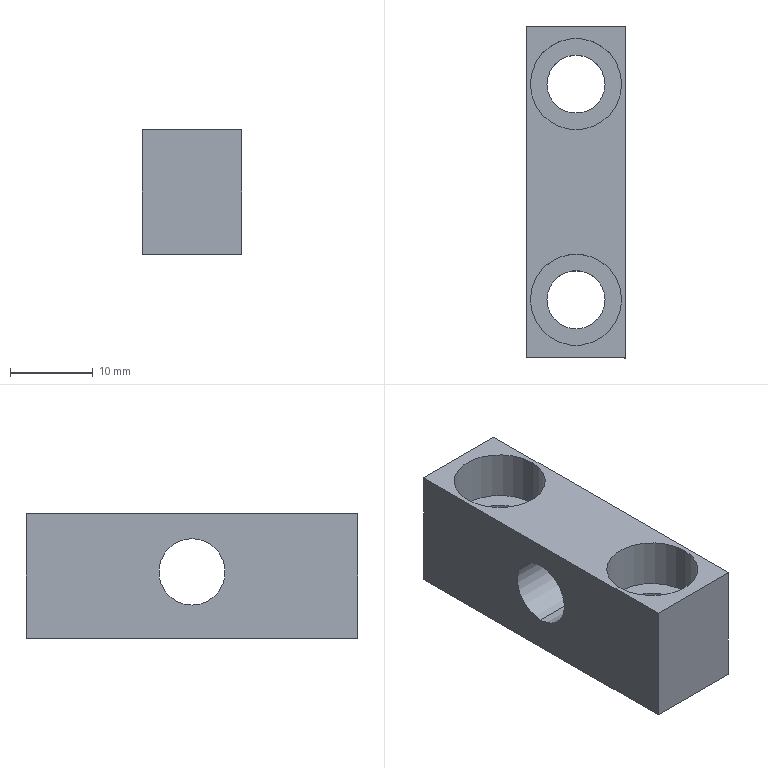Component | SolidWorks | -BeltTensionBlock-1 | 1 solid | 18 faces | box 12 x 40 x 15 mm | volume 4764 mm3 | cylinder 10 | plane 8 | commonest cylinder face diameters 11 x4 7 x4 8 x2
build123d program:
from build123d import *

# Parameters (mm, degrees)
SKETCH1_W                                           = 15
SKETCH1_H                                           = 40
BOSS_EXTRUDE1_DEPTH                                 = 12
SKETCH2_R                                           = 4
CUT_EXTRUDE1_DEPTH                                  = 12
CYLINDRICAL_COUNTERSUNK_HOLE_FOR_M6_HEX_D           = 7
CYLINDRICAL_COUNTERSUNK_HOLE_FOR_M6_HEX_CBORE_D     = 11
CYLINDRICAL_COUNTERSUNK_HOLE_FOR_M6_HEX_CBORE_DEPTH = 6


with BuildPart() as part:
    # Sketch1 → Boss-Extrude1 (new body)
    with BuildSketch(Plane.XY):
        Rectangle(SKETCH1_W, SKETCH1_H)
    extrude(amount=BOSS_EXTRUDE1_DEPTH)

    # Sketch2 → Cut-Extrude1 (cut)
    with BuildSketch(Plane.XY.offset(12)):
        with Locations((0.5, 0)):
            Circle(SKETCH2_R)
    extrude(amount=-CUT_EXTRUDE1_DEPTH, mode=Mode.SUBTRACT)

    # Cylindrical Countersunk Hole for M6 Hex (through all)
    with Locations(Plane(origin=(7.5, 0, 0), x_dir=(0, 0, -1), z_dir=(1, 0, 0))):
        with Locations((-6, 13), (-6, -13)):
            CounterBoreHole(CYLINDRICAL_COUNTERSUNK_HOLE_FOR_M6_HEX_D / 2, CYLINDRICAL_COUNTERSUNK_HOLE_FOR_M6_HEX_CBORE_D / 2, CYLINDRICAL_COUNTERSUNK_HOLE_FOR_M6_HEX_CBORE_DEPTH)


solid = part.part

# Placed as in the assembly
solid = solid.moved(Location((-178, 1094.5, 159.5), (0, -90, 0)))
STEP:
#1=COLOUR_RGB('',0.7922,0.8196,0.9333);
#2=FILL_AREA_STYLE_COLOUR('',#1);
#3=FILL_AREA_STYLE('',(#2));
#4=SURFACE_STYLE_FILL_AREA(#3);
#5=SURFACE_SIDE_STYLE('',(#4));
#6=SURFACE_STYLE_USAGE(.BOTH.,#5);
#7=PRESENTATION_STYLE_ASSIGNMENT((#6));
#8=CARTESIAN_POINT('',(-7.461,43.602,6.339));
#9=VERTEX_POINT('',#8);
#10=CARTESIAN_POINT('',(-7.028,43.602,6.339));
#11=VERTEX_POINT('',#10);
#12=CARTESIAN_POINT('',(-7.244,43.602,6.339));
#13=DIRECTION('',(0.,-0.,1.));
#14=DIRECTION('',(1.,0.,0.));
#15=AXIS2_PLACEMENT_3D('',#12,#13,#14);
#16=CIRCLE('',#15,0.2165);
#17=EDGE_CURVE('',#9,#11,#16,.T.);
#18=ORIENTED_EDGE('',*,*,#17,.F.);
#19=CARTESIAN_POINT('',(-7.461,43.602,6.575));
#20=VERTEX_POINT('',#19);
#21=CARTESIAN_POINT('',(-7.461,43.602,6.575));
#22=DIRECTION('',(0.,-0.,1.));
#23=VECTOR('',#22,39.37);
#24=LINE('',#21,#23);
#25=EDGE_CURVE('',#9,#20,#24,.T.);
#26=ORIENTED_EDGE('',*,*,#25,.T.);
#27=CARTESIAN_POINT('',(-7.028,43.602,6.575));
#28=VERTEX_POINT('',#27);
#29=CARTESIAN_POINT('',(-7.244,43.602,6.575));
#30=DIRECTION('',(0.,-0.,1.));
#31=DIRECTION('',(1.,0.,0.));
#32=AXIS2_PLACEMENT_3D('',#29,#30,#31);
#33=CIRCLE('',#32,0.2165);
#34=EDGE_CURVE('',#20,#28,#33,.T.);
#35=ORIENTED_EDGE('',*,*,#34,.T.);
#36=CARTESIAN_POINT('',(-7.028,43.602,6.575));
#37=DIRECTION('',(0.,-0.,1.));
#38=VECTOR('',#37,39.37);
#39=LINE('',#36,#38);
#40=EDGE_CURVE('',#11,#28,#39,.T.);
#41=ORIENTED_EDGE('',*,*,#40,.F.);
#42=EDGE_LOOP('',(#18,#26,#35,#41));
#43=FACE_OUTER_BOUND('',#42,.T.);
#44=CARTESIAN_POINT('',(-7.244,43.602,6.575));
#45=DIRECTION('',(0.,-0.,1.));
#46=DIRECTION('',(1.,0.,0.));
#47=AXIS2_PLACEMENT_3D('',#44,#45,#46);
#48=CYLINDRICAL_SURFACE('',#47,0.2165);
#49=ADVANCED_FACE('',(#43),#48,.F.);
#50=CARTESIAN_POINT('',(-7.382,43.602,5.984));
#51=VERTEX_POINT('',#50);
#52=CARTESIAN_POINT('',(-7.106,43.602,5.984));
#53=VERTEX_POINT('',#52);
#54=CARTESIAN_POINT('',(-7.244,43.602,5.984));
#55=DIRECTION('',(0.,-0.,1.));
#56=DIRECTION('',(1.,0.,0.));
#57=AXIS2_PLACEMENT_3D('',#54,#55,#56);
#58=CIRCLE('',#57,0.1378);
#59=EDGE_CURVE('',#51,#53,#58,.T.);
#60=ORIENTED_EDGE('',*,*,#59,.F.);
#61=CARTESIAN_POINT('',(-7.382,43.602,6.339));
#62=VERTEX_POINT('',#61);
#63=CARTESIAN_POINT('',(-7.382,43.602,6.575));
#64=DIRECTION('',(0.,-0.,1.));
#65=VECTOR('',#64,39.37);
#66=LINE('',#63,#65);
#67=EDGE_CURVE('',#51,#62,#66,.T.);
#68=ORIENTED_EDGE('',*,*,#67,.T.);
#69=CARTESIAN_POINT('',(-7.106,43.602,6.339));
#70=VERTEX_POINT('',#69);
#71=CARTESIAN_POINT('',(-7.244,43.602,6.339));
#72=DIRECTION('',(0.,-0.,1.));
#73=DIRECTION('',(1.,0.,0.));
#74=AXIS2_PLACEMENT_3D('',#71,#72,#73);
#75=CIRCLE('',#74,0.1378);
#76=EDGE_CURVE('',#62,#70,#75,.T.);
#77=ORIENTED_EDGE('',*,*,#76,.T.);
#78=CARTESIAN_POINT('',(-7.106,43.602,6.575));
#79=DIRECTION('',(0.,-0.,1.));
#80=VECTOR('',#79,39.37);
#81=LINE('',#78,#80);
#82=EDGE_CURVE('',#53,#70,#81,.T.);
#83=ORIENTED_EDGE('',*,*,#82,.F.);
#84=EDGE_LOOP('',(#60,#68,#77,#83));
#85=FACE_OUTER_BOUND('',#84,.T.);
#86=CARTESIAN_POINT('',(-7.244,43.602,6.575));
#87=DIRECTION('',(0.,-0.,1.));
#88=DIRECTION('',(1.,0.,0.));
#89=AXIS2_PLACEMENT_3D('',#86,#87,#88);
#90=CYLINDRICAL_SURFACE('',#89,0.1378);
#91=ADVANCED_FACE('',(#85),#90,.F.);
#92=CARTESIAN_POINT('',(-7.461,42.579,6.339));
#93=VERTEX_POINT('',#92);
#94=CARTESIAN_POINT('',(-7.028,42.579,6.339));
#95=VERTEX_POINT('',#94);
#96=CARTESIAN_POINT('',(-7.244,42.579,6.339));
#97=DIRECTION('',(0.,-0.,1.));
#98=DIRECTION('',(1.,0.,0.));
#99=AXIS2_PLACEMENT_3D('',#96,#97,#98);
#100=CIRCLE('',#99,0.2165);
#101=EDGE_CURVE('',#93,#95,#100,.T.);
#102=ORIENTED_EDGE('',*,*,#101,.F.);
#103=CARTESIAN_POINT('',(-7.461,42.579,6.575));
#104=VERTEX_POINT('',#103);
#105=CARTESIAN_POINT('',(-7.461,42.579,6.575));
#106=DIRECTION('',(0.,-0.,1.));
#107=VECTOR('',#106,39.37);
#108=LINE('',#105,#107);
#109=EDGE_CURVE('',#93,#104,#108,.T.);
#110=ORIENTED_EDGE('',*,*,#109,.T.);
#111=CARTESIAN_POINT('',(-7.028,42.579,6.575));
#112=VERTEX_POINT('',#111);
#113=CARTESIAN_POINT('',(-7.244,42.579,6.575));
#114=DIRECTION('',(0.,-0.,1.));
#115=DIRECTION('',(1.,0.,0.));
#116=AXIS2_PLACEMENT_3D('',#113,#114,#115);
#117=CIRCLE('',#116,0.2165);
#118=EDGE_CURVE('',#104,#112,#117,.T.);
#119=ORIENTED_EDGE('',*,*,#118,.T.);
#120=CARTESIAN_POINT('',(-7.028,42.579,6.575));
#121=DIRECTION('',(0.,-0.,1.));
#122=VECTOR('',#121,39.37);
#123=LINE('',#120,#122);
#124=EDGE_CURVE('',#95,#112,#123,.T.);
#125=ORIENTED_EDGE('',*,*,#124,.F.);
#126=EDGE_LOOP('',(#102,#110,#119,#125));
#127=FACE_OUTER_BOUND('',#126,.T.);
#128=CARTESIAN_POINT('',(-7.244,42.579,6.575));
#129=DIRECTION('',(0.,-0.,1.));
#130=DIRECTION('',(1.,0.,0.));
#131=AXIS2_PLACEMENT_3D('',#128,#129,#130);
#132=CYLINDRICAL_SURFACE('',#131,0.2165);
#133=ADVANCED_FACE('',(#127),#132,.F.);
#134=CARTESIAN_POINT('',(-7.382,42.579,5.984));
#135=VERTEX_POINT('',#134);
#136=CARTESIAN_POINT('',(-7.106,42.579,5.984));
#137=VERTEX_POINT('',#136);
#138=CARTESIAN_POINT('',(-7.244,42.579,5.984));
#139=DIRECTION('',(0.,-0.,1.));
#140=DIRECTION('',(1.,0.,0.));
#141=AXIS2_PLACEMENT_3D('',#138,#139,#140);
#142=CIRCLE('',#141,0.1378);
#143=EDGE_CURVE('',#135,#137,#142,.T.);
#144=ORIENTED_EDGE('',*,*,#143,.F.);
#145=CARTESIAN_POINT('',(-7.382,42.579,6.339));
#146=VERTEX_POINT('',#145);
#147=CARTESIAN_POINT('',(-7.382,42.579,6.575));
#148=DIRECTION('',(0.,-0.,1.));
#149=VECTOR('',#148,39.37);
#150=LINE('',#147,#149);
#151=EDGE_CURVE('',#135,#146,#150,.T.);
#152=ORIENTED_EDGE('',*,*,#151,.T.);
#153=CARTESIAN_POINT('',(-7.106,42.579,6.339));
#154=VERTEX_POINT('',#153);
#155=CARTESIAN_POINT('',(-7.244,42.579,6.339));
#156=DIRECTION('',(0.,-0.,1.));
#157=DIRECTION('',(1.,0.,0.));
#158=AXIS2_PLACEMENT_3D('',#155,#156,#157);
#159=CIRCLE('',#158,0.1378);
#160=EDGE_CURVE('',#146,#154,#159,.T.);
#161=ORIENTED_EDGE('',*,*,#160,.T.);
#162=CARTESIAN_POINT('',(-7.106,42.579,6.575));
#163=DIRECTION('',(0.,-0.,1.));
#164=VECTOR('',#163,39.37);
#165=LINE('',#162,#164);
#166=EDGE_CURVE('',#137,#154,#165,.T.);
#167=ORIENTED_EDGE('',*,*,#166,.F.);
#168=EDGE_LOOP('',(#144,#152,#161,#167));
#169=FACE_OUTER_BOUND('',#168,.T.);
#170=CARTESIAN_POINT('',(-7.244,42.579,6.575));
#171=DIRECTION('',(0.,-0.,1.));
#172=DIRECTION('',(1.,0.,0.));
#173=AXIS2_PLACEMENT_3D('',#170,#171,#172);
#174=CYLINDRICAL_SURFACE('',#173,0.1378);
#175=ADVANCED_FACE('',(#169),#174,.F.);
#176=CARTESIAN_POINT('',(-7.008,43.091,6.142));
#177=VERTEX_POINT('',#176);
#178=CARTESIAN_POINT('',(-7.008,43.091,6.457));
#179=VERTEX_POINT('',#178);
#180=CARTESIAN_POINT('',(-7.008,43.091,6.299));
#181=DIRECTION('',(-1.,0.,0.));
#182=DIRECTION('',(0.,0.,1.));
#183=AXIS2_PLACEMENT_3D('',#180,#181,#182);
#184=CIRCLE('',#183,0.1575);
#185=EDGE_CURVE('',#177,#179,#184,.T.);
#186=ORIENTED_EDGE('',*,*,#185,.F.);
#187=CARTESIAN_POINT('',(-7.48,43.091,6.142));
#188=VERTEX_POINT('',#187);
#189=CARTESIAN_POINT('',(-7.008,43.091,6.142));
#190=DIRECTION('',(-1.,0.,0.));
#191=VECTOR('',#190,39.37);
#192=LINE('',#189,#191);
#193=EDGE_CURVE('',#177,#188,#192,.T.);
#194=ORIENTED_EDGE('',*,*,#193,.T.);
#195=CARTESIAN_POINT('',(-7.48,43.091,6.457));
#196=VERTEX_POINT('',#195);
#197=CARTESIAN_POINT('',(-7.48,43.091,6.299));
#198=DIRECTION('',(-1.,0.,0.));
#199=DIRECTION('',(0.,0.,1.));
#200=AXIS2_PLACEMENT_3D('',#197,#198,#199);
#201=CIRCLE('',#200,0.1575);
#202=EDGE_CURVE('',#188,#196,#201,.T.);
#203=ORIENTED_EDGE('',*,*,#202,.T.);
#204=CARTESIAN_POINT('',(-7.008,43.091,6.457));
#205=DIRECTION('',(-1.,0.,0.));
#206=VECTOR('',#205,39.37);
#207=LINE('',#204,#206);
#208=EDGE_CURVE('',#179,#196,#207,.T.);
#209=ORIENTED_EDGE('',*,*,#208,.F.);
#210=EDGE_LOOP('',(#186,#194,#203,#209));
#211=FACE_OUTER_BOUND('',#210,.T.);
#212=CARTESIAN_POINT('',(-7.008,43.091,6.299));
#213=DIRECTION('',(-1.,0.,0.));
#214=DIRECTION('',(0.,0.,1.));
#215=AXIS2_PLACEMENT_3D('',#212,#213,#214);
#216=CYLINDRICAL_SURFACE('',#215,0.1575);
#217=ADVANCED_FACE('',(#211),#216,.F.);
#218=CARTESIAN_POINT('',(-7.244,43.602,6.575));
#219=DIRECTION('',(0.,-0.,1.));
#220=DIRECTION('',(1.,0.,0.));
#221=AXIS2_PLACEMENT_3D('',#218,#219,#220);
#222=CIRCLE('',#221,0.2165);
#223=EDGE_CURVE('',#28,#20,#222,.T.);
#224=ORIENTED_EDGE('',*,*,#223,.F.);
#225=ORIENTED_EDGE('',*,*,#34,.F.);
#226=EDGE_LOOP('',(#224,#225));
#227=FACE_BOUND('',#226,.T.);
#228=CARTESIAN_POINT('',(-7.244,42.579,6.575));
#229=DIRECTION('',(0.,-0.,1.));
#230=DIRECTION('',(1.,0.,0.));
#231=AXIS2_PLACEMENT_3D('',#228,#229,#230);
#232=CIRCLE('',#231,0.2165);
#233=EDGE_CURVE('',#112,#104,#232,.T.);
#234=ORIENTED_EDGE('',*,*,#233,.F.);
#235=ORIENTED_EDGE('',*,*,#118,.F.);
#236=EDGE_LOOP('',(#234,#235));
#237=FACE_BOUND('',#236,.T.);
#238=CARTESIAN_POINT('',(-7.008,42.303,6.575));
#239=VERTEX_POINT('',#238);
#240=CARTESIAN_POINT('',(-7.008,43.878,6.575));
#241=VERTEX_POINT('',#240);
#242=CARTESIAN_POINT('',(-7.008,43.878,6.575));
#243=DIRECTION('',(0.,1.,0.));
#244=VECTOR('',#243,39.37);
#245=LINE('',#242,#244);
#246=EDGE_CURVE('',#239,#241,#245,.T.);
#247=ORIENTED_EDGE('',*,*,#246,.T.);
#248=CARTESIAN_POINT('',(-7.48,43.878,6.575));
#249=VERTEX_POINT('',#248);
#250=CARTESIAN_POINT('',(-7.48,43.878,6.575));
#251=DIRECTION('',(1.,-0.,-0.));
#252=VECTOR('',#251,39.37);
#253=LINE('',#250,#252);
#254=EDGE_CURVE('',#249,#241,#253,.T.);
#255=ORIENTED_EDGE('',*,*,#254,.F.);
#256=CARTESIAN_POINT('',(-7.48,42.303,6.575));
#257=VERTEX_POINT('',#256);
#258=CARTESIAN_POINT('',(-7.48,43.878,6.575));
#259=DIRECTION('',(0.,1.,0.));
#260=VECTOR('',#259,39.37);
#261=LINE('',#258,#260);
#262=EDGE_CURVE('',#257,#249,#261,.T.);
#263=ORIENTED_EDGE('',*,*,#262,.F.);
#264=CARTESIAN_POINT('',(-7.48,42.303,6.575));
#265=DIRECTION('',(1.,-0.,-0.));
#266=VECTOR('',#265,39.37);
#267=LINE('',#264,#266);
#268=EDGE_CURVE('',#257,#239,#267,.T.);
#269=ORIENTED_EDGE('',*,*,#268,.T.);
#270=EDGE_LOOP('',(#247,#255,#263,#269));
#271=FACE_OUTER_BOUND('',#270,.T.);
#272=CARTESIAN_POINT('',(-7.48,43.878,6.575));
#273=DIRECTION('',(-0.,0.,-1.));
#274=DIRECTION('',(-0.,-1.,-0.));
#275=AXIS2_PLACEMENT_3D('',#272,#273,#274);
#276=PLANE('',#275);
#277=ADVANCED_FACE('',(#227,#237,#271),#276,.F.);
#278=CARTESIAN_POINT('',(-7.008,43.878,5.984));
#279=VERTEX_POINT('',#278);
#280=CARTESIAN_POINT('',(-7.008,43.878,5.984));
#281=DIRECTION('',(-0.,0.,-1.));
#282=VECTOR('',#281,39.37);
#283=LINE('',#280,#282);
#284=EDGE_CURVE('',#241,#279,#283,.T.);
#285=ORIENTED_EDGE('',*,*,#284,.T.);
#286=CARTESIAN_POINT('',(-7.48,43.878,5.984));
#287=VERTEX_POINT('',#286);
#288=CARTESIAN_POINT('',(-7.48,43.878,5.984));
#289=DIRECTION('',(1.,-0.,-0.));
#290=VECTOR('',#289,39.37);
#291=LINE('',#288,#290);
#292=EDGE_CURVE('',#287,#279,#291,.T.);
#293=ORIENTED_EDGE('',*,*,#292,.F.);
#294=CARTESIAN_POINT('',(-7.48,43.878,5.984));
#295=DIRECTION('',(-0.,0.,-1.));
#296=VECTOR('',#295,39.37);
#297=LINE('',#294,#296);
#298=EDGE_CURVE('',#249,#287,#297,.T.);
#299=ORIENTED_EDGE('',*,*,#298,.F.);
#300=ORIENTED_EDGE('',*,*,#254,.T.);
#301=EDGE_LOOP('',(#285,#293,#299,#300));
#302=FACE_OUTER_BOUND('',#301,.T.);
#303=CARTESIAN_POINT('',(-7.48,43.878,5.984));
#304=DIRECTION('',(-0.,-1.,-0.));
#305=DIRECTION('',(1.,-0.,-0.));
#306=AXIS2_PLACEMENT_3D('',#303,#304,#305);
#307=PLANE('',#306);
#308=ADVANCED_FACE('',(#302),#307,.F.);
#309=CARTESIAN_POINT('',(-7.244,43.602,5.984));
#310=DIRECTION('',(0.,-0.,1.));
#311=DIRECTION('',(1.,0.,0.));
#312=AXIS2_PLACEMENT_3D('',#309,#310,#311);
#313=CIRCLE('',#312,0.1378);
#314=EDGE_CURVE('',#53,#51,#313,.T.);
#315=ORIENTED_EDGE('',*,*,#314,.T.);
#316=ORIENTED_EDGE('',*,*,#59,.T.);
#317=EDGE_LOOP('',(#315,#316));
#318=FACE_BOUND('',#317,.T.);
#319=CARTESIAN_POINT('',(-7.244,42.579,5.984));
#320=DIRECTION('',(0.,-0.,1.));
#321=DIRECTION('',(1.,0.,0.));
#322=AXIS2_PLACEMENT_3D('',#319,#320,#321);
#323=CIRCLE('',#322,0.1378);
#324=EDGE_CURVE('',#137,#135,#323,.T.);
#325=ORIENTED_EDGE('',*,*,#324,.T.);
#326=ORIENTED_EDGE('',*,*,#143,.T.);
#327=EDGE_LOOP('',(#325,#326));
#328=FACE_BOUND('',#327,.T.);
#329=CARTESIAN_POINT('',(-7.008,42.303,5.984));
#330=VERTEX_POINT('',#329);
#331=CARTESIAN_POINT('',(-7.008,43.878,5.984));
#332=DIRECTION('',(-0.,-1.,-0.));
#333=VECTOR('',#332,39.37);
#334=LINE('',#331,#333);
#335=EDGE_CURVE('',#279,#330,#334,.T.);
#336=ORIENTED_EDGE('',*,*,#335,.T.);
#337=CARTESIAN_POINT('',(-7.48,42.303,5.984));
#338=VERTEX_POINT('',#337);
#339=CARTESIAN_POINT('',(-7.48,42.303,5.984));
#340=DIRECTION('',(1.,-0.,-0.));
#341=VECTOR('',#340,39.37);
#342=LINE('',#339,#341);
#343=EDGE_CURVE('',#338,#330,#342,.T.);
#344=ORIENTED_EDGE('',*,*,#343,.F.);
#345=CARTESIAN_POINT('',(-7.48,43.878,5.984));
#346=DIRECTION('',(-0.,-1.,-0.));
#347=VECTOR('',#346,39.37);
#348=LINE('',#345,#347);
#349=EDGE_CURVE('',#287,#338,#348,.T.);
#350=ORIENTED_EDGE('',*,*,#349,.F.);
#351=ORIENTED_EDGE('',*,*,#292,.T.);
#352=EDGE_LOOP('',(#336,#344,#350,#351));
#353=FACE_OUTER_BOUND('',#352,.T.);
#354=CARTESIAN_POINT('',(-7.48,43.878,5.984));
#355=DIRECTION('',(0.,-0.,1.));
#356=DIRECTION('',(0.,1.,0.));
#357=AXIS2_PLACEMENT_3D('',#354,#355,#356);
#358=PLANE('',#357);
#359=ADVANCED_FACE('',(#318,#328,#353),#358,.F.);
#360=CARTESIAN_POINT('',(-7.008,42.303,5.984));
#361=DIRECTION('',(0.,-0.,1.));
#362=VECTOR('',#361,39.37);
#363=LINE('',#360,#362);
#364=EDGE_CURVE('',#330,#239,#363,.T.);
#365=ORIENTED_EDGE('',*,*,#364,.T.);
#366=ORIENTED_EDGE('',*,*,#268,.F.);
#367=CARTESIAN_POINT('',(-7.48,42.303,5.984));
#368=DIRECTION('',(0.,-0.,1.));
#369=VECTOR('',#368,39.37);
#370=LINE('',#367,#369);
#371=EDGE_CURVE('',#338,#257,#370,.T.);
#372=ORIENTED_EDGE('',*,*,#371,.F.);
#373=ORIENTED_EDGE('',*,*,#343,.T.);
#374=EDGE_LOOP('',(#365,#366,#372,#373));
#375=FACE_OUTER_BOUND('',#374,.T.);
#376=CARTESIAN_POINT('',(-7.48,42.303,5.984));
#377=DIRECTION('',(0.,1.,0.));
#378=DIRECTION('',(-1.,0.,0.));
#379=AXIS2_PLACEMENT_3D('',#376,#377,#378);
#380=PLANE('',#379);
#381=ADVANCED_FACE('',(#375),#380,.F.);
#382=CARTESIAN_POINT('',(-7.48,43.091,6.299));
#383=DIRECTION('',(-1.,0.,0.));
#384=DIRECTION('',(0.,0.,1.));
#385=AXIS2_PLACEMENT_3D('',#382,#383,#384);
#386=CIRCLE('',#385,0.1575);
#387=EDGE_CURVE('',#196,#188,#386,.T.);
#388=ORIENTED_EDGE('',*,*,#387,.F.);
#389=ORIENTED_EDGE('',*,*,#202,.F.);
#390=EDGE_LOOP('',(#388,#389));
#391=FACE_BOUND('',#390,.T.);
#392=ORIENTED_EDGE('',*,*,#262,.T.);
#393=ORIENTED_EDGE('',*,*,#298,.T.);
#394=ORIENTED_EDGE('',*,*,#349,.T.);
#395=ORIENTED_EDGE('',*,*,#371,.T.);
#396=EDGE_LOOP('',(#392,#393,#394,#395));
#397=FACE_OUTER_BOUND('',#396,.T.);
#398=CARTESIAN_POINT('',(-7.48,43.091,6.28));
#399=DIRECTION('',(-1.,0.,0.));
#400=DIRECTION('',(0.,-0.,1.));
#401=AXIS2_PLACEMENT_3D('',#398,#399,#400);
#402=PLANE('',#401);
#403=ADVANCED_FACE('',(#391,#397),#402,.T.);
#404=CARTESIAN_POINT('',(-7.008,43.091,6.299));
#405=DIRECTION('',(-1.,0.,0.));
#406=DIRECTION('',(0.,0.,1.));
#407=AXIS2_PLACEMENT_3D('',#404,#405,#406);
#408=CIRCLE('',#407,0.1575);
#409=EDGE_CURVE('',#179,#177,#408,.T.);
#410=ORIENTED_EDGE('',*,*,#409,.T.);
#411=ORIENTED_EDGE('',*,*,#185,.T.);
#412=EDGE_LOOP('',(#410,#411));
#413=FACE_BOUND('',#412,.T.);
#414=ORIENTED_EDGE('',*,*,#246,.F.);
#415=ORIENTED_EDGE('',*,*,#364,.F.);
#416=ORIENTED_EDGE('',*,*,#335,.F.);
#417=ORIENTED_EDGE('',*,*,#284,.F.);
#418=EDGE_LOOP('',(#414,#415,#416,#417));
#419=FACE_OUTER_BOUND('',#418,.T.);
#420=CARTESIAN_POINT('',(-7.008,43.091,6.28));
#421=DIRECTION('',(-1.,0.,0.));
#422=DIRECTION('',(0.,-0.,1.));
#423=AXIS2_PLACEMENT_3D('',#420,#421,#422);
#424=PLANE('',#423);
#425=ADVANCED_FACE('',(#413,#419),#424,.F.);
#426=ORIENTED_EDGE('',*,*,#193,.F.);
#427=ORIENTED_EDGE('',*,*,#409,.F.);
#428=ORIENTED_EDGE('',*,*,#208,.T.);
#429=ORIENTED_EDGE('',*,*,#387,.T.);
#430=EDGE_LOOP('',(#426,#427,#428,#429));
#431=FACE_OUTER_BOUND('',#430,.T.);
#432=CARTESIAN_POINT('',(-7.008,43.091,6.299));
#433=DIRECTION('',(-1.,0.,0.));
#434=DIRECTION('',(0.,0.,1.));
#435=AXIS2_PLACEMENT_3D('',#432,#433,#434);
#436=CYLINDRICAL_SURFACE('',#435,0.1575);
#437=ADVANCED_FACE('',(#431),#436,.F.);
#438=ORIENTED_EDGE('',*,*,#151,.F.);
#439=ORIENTED_EDGE('',*,*,#324,.F.);
#440=ORIENTED_EDGE('',*,*,#166,.T.);
#441=CARTESIAN_POINT('',(-7.244,42.579,6.339));
#442=DIRECTION('',(0.,-0.,1.));
#443=DIRECTION('',(1.,0.,0.));
#444=AXIS2_PLACEMENT_3D('',#441,#442,#443);
#445=CIRCLE('',#444,0.1378);
#446=EDGE_CURVE('',#154,#146,#445,.T.);
#447=ORIENTED_EDGE('',*,*,#446,.T.);
#448=EDGE_LOOP('',(#438,#439,#440,#447));
#449=FACE_OUTER_BOUND('',#448,.T.);
#450=CARTESIAN_POINT('',(-7.244,42.579,6.575));
#451=DIRECTION('',(0.,-0.,1.));
#452=DIRECTION('',(1.,0.,0.));
#453=AXIS2_PLACEMENT_3D('',#450,#451,#452);
#454=CYLINDRICAL_SURFACE('',#453,0.1378);
#455=ADVANCED_FACE('',(#449),#454,.F.);
#456=ORIENTED_EDGE('',*,*,#446,.F.);
#457=ORIENTED_EDGE('',*,*,#160,.F.);
#458=EDGE_LOOP('',(#456,#457));
#459=FACE_BOUND('',#458,.T.);
#460=CARTESIAN_POINT('',(-7.244,42.579,6.339));
#461=DIRECTION('',(0.,-0.,1.));
#462=DIRECTION('',(1.,0.,0.));
#463=AXIS2_PLACEMENT_3D('',#460,#461,#462);
#464=CIRCLE('',#463,0.2165);
#465=EDGE_CURVE('',#95,#93,#464,.T.);
#466=ORIENTED_EDGE('',*,*,#465,.T.);
#467=ORIENTED_EDGE('',*,*,#101,.T.);
#468=EDGE_LOOP('',(#466,#467));
#469=FACE_OUTER_BOUND('',#468,.T.);
#470=CARTESIAN_POINT('',(-7.244,42.717,6.339));
#471=DIRECTION('',(0.,0.,-1.));
#472=DIRECTION('',(-1.,0.,0.));
#473=AXIS2_PLACEMENT_3D('',#470,#471,#472);
#474=PLANE('',#473);
#475=ADVANCED_FACE('',(#459,#469),#474,.F.);
#476=ORIENTED_EDGE('',*,*,#109,.F.);
#477=ORIENTED_EDGE('',*,*,#465,.F.);
#478=ORIENTED_EDGE('',*,*,#124,.T.);
#479=ORIENTED_EDGE('',*,*,#233,.T.);
#480=EDGE_LOOP('',(#476,#477,#478,#479));
#481=FACE_OUTER_BOUND('',#480,.T.);
#482=CARTESIAN_POINT('',(-7.244,42.579,6.575));
#483=DIRECTION('',(0.,-0.,1.));
#484=DIRECTION('',(1.,0.,0.));
#485=AXIS2_PLACEMENT_3D('',#482,#483,#484);
#486=CYLINDRICAL_SURFACE('',#485,0.2165);
#487=ADVANCED_FACE('',(#481),#486,.F.);
#488=ORIENTED_EDGE('',*,*,#67,.F.);
#489=ORIENTED_EDGE('',*,*,#314,.F.);
#490=ORIENTED_EDGE('',*,*,#82,.T.);
#491=CARTESIAN_POINT('',(-7.244,43.602,6.339));
#492=DIRECTION('',(0.,-0.,1.));
#493=DIRECTION('',(1.,0.,0.));
#494=AXIS2_PLACEMENT_3D('',#491,#492,#493);
#495=CIRCLE('',#494,0.1378);
#496=EDGE_CURVE('',#70,#62,#495,.T.);
#497=ORIENTED_EDGE('',*,*,#496,.T.);
#498=EDGE_LOOP('',(#488,#489,#490,#497));
#499=FACE_OUTER_BOUND('',#498,.T.);
#500=CARTESIAN_POINT('',(-7.244,43.602,6.575));
#501=DIRECTION('',(0.,-0.,1.));
#502=DIRECTION('',(1.,0.,0.));
#503=AXIS2_PLACEMENT_3D('',#500,#501,#502);
#504=CYLINDRICAL_SURFACE('',#503,0.1378);
#505=ADVANCED_FACE('',(#499),#504,.F.);
#506=ORIENTED_EDGE('',*,*,#496,.F.);
#507=ORIENTED_EDGE('',*,*,#76,.F.);
#508=EDGE_LOOP('',(#506,#507));
#509=FACE_BOUND('',#508,.T.);
#510=CARTESIAN_POINT('',(-7.244,43.602,6.339));
#511=DIRECTION('',(0.,-0.,1.));
#512=DIRECTION('',(1.,0.,0.));
#513=AXIS2_PLACEMENT_3D('',#510,#511,#512);
#514=CIRCLE('',#513,0.2165);
#515=EDGE_CURVE('',#11,#9,#514,.T.);
#516=ORIENTED_EDGE('',*,*,#515,.T.);
#517=ORIENTED_EDGE('',*,*,#17,.T.);
#518=EDGE_LOOP('',(#516,#517));
#519=FACE_OUTER_BOUND('',#518,.T.);
#520=CARTESIAN_POINT('',(-7.244,43.74,6.339));
#521=DIRECTION('',(0.,0.,-1.));
#522=DIRECTION('',(-1.,0.,0.));
#523=AXIS2_PLACEMENT_3D('',#520,#521,#522);
#524=PLANE('',#523);
#525=ADVANCED_FACE('',(#509,#519),#524,.F.);
#526=ORIENTED_EDGE('',*,*,#25,.F.);
#527=ORIENTED_EDGE('',*,*,#515,.F.);
#528=ORIENTED_EDGE('',*,*,#40,.T.);
#529=ORIENTED_EDGE('',*,*,#223,.T.);
#530=EDGE_LOOP('',(#526,#527,#528,#529));
#531=FACE_OUTER_BOUND('',#530,.T.);
#532=CARTESIAN_POINT('',(-7.244,43.602,6.575));
#533=DIRECTION('',(0.,-0.,1.));
#534=DIRECTION('',(1.,0.,0.));
#535=AXIS2_PLACEMENT_3D('',#532,#533,#534);
#536=CYLINDRICAL_SURFACE('',#535,0.2165);
#537=ADVANCED_FACE('',(#531),#536,.F.);
#538=CLOSED_SHELL('',(#49,#91,#133,#175,#217,#277,#308,#359,#381,#403,#425,#437,#455,#475,#487,#505,#525,#537));
#539=MANIFOLD_SOLID_BREP('',#538);
#540=STYLED_ITEM('',(#7),#539);
#541=(LENGTH_UNIT()NAMED_UNIT(*)SI_UNIT($,.METRE.));
#542=LENGTH_MEASURE_WITH_UNIT(LENGTH_MEASURE(0.0254),#541);
#543=DIMENSIONAL_EXPONENTS(1.,0.,0.,0.,0.,0.,0.);
#544=(CONVERSION_BASED_UNIT('',#542)LENGTH_UNIT()NAMED_UNIT(#543));
#545=UNCERTAINTY_MEASURE_WITH_UNIT(LENGTH_MEASURE(0.00001),#544,'','');
#546=(NAMED_UNIT(*)PLANE_ANGLE_UNIT()SI_UNIT($,.RADIAN.));
#547=(NAMED_UNIT(*)SI_UNIT($,.STERADIAN.)SOLID_ANGLE_UNIT());
#548=(GEOMETRIC_REPRESENTATION_CONTEXT(3)GLOBAL_UNCERTAINTY_ASSIGNED_CONTEXT((#545))GLOBAL_UNIT_ASSIGNED_CONTEXT((#544,#546,#547))REPRESENTATION_CONTEXT('',''));
#549=MECHANICAL_DESIGN_GEOMETRIC_PRESENTATION_REPRESENTATION('',(#540),#548);
#550=CARTESIAN_POINT('',(0.,0.,0.));
#551=DIRECTION('',(0.,0.,1.));
#552=DIRECTION('',(1.,0.,0.));
#553=AXIS2_PLACEMENT_3D('',#550,#551,#552);
#554=(LENGTH_UNIT()NAMED_UNIT(*)SI_UNIT($,.METRE.));
#555=LENGTH_MEASURE_WITH_UNIT(LENGTH_MEASURE(0.0254),#554);
#556=DIMENSIONAL_EXPONENTS(1.,0.,0.,0.,0.,0.,0.);
#557=(CONVERSION_BASED_UNIT('',#555)LENGTH_UNIT()NAMED_UNIT(#556));
#558=UNCERTAINTY_MEASURE_WITH_UNIT(LENGTH_MEASURE(0.00001),#557,'','');
#559=(NAMED_UNIT(*)PLANE_ANGLE_UNIT()SI_UNIT($,.RADIAN.));
#560=(NAMED_UNIT(*)SI_UNIT($,.STERADIAN.)SOLID_ANGLE_UNIT());
#561=(GEOMETRIC_REPRESENTATION_CONTEXT(3)GLOBAL_UNCERTAINTY_ASSIGNED_CONTEXT((#558))GLOBAL_UNIT_ASSIGNED_CONTEXT((#557,#559,#560))REPRESENTATION_CONTEXT('',''));
#562=ADVANCED_BREP_SHAPE_REPRESENTATION('',(#539,#553),#561);
#563=PRESENTATION_LAYER_ASSIGNMENT('','',(#540));